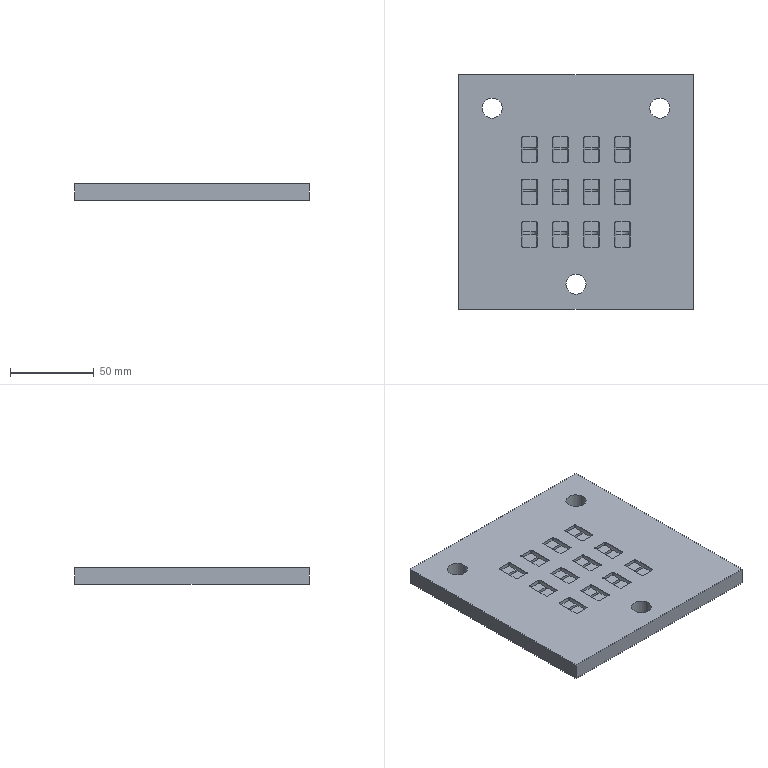CAM job | NX | mm | 3-axis | 1 set-up | 3 operations | part box 140 x 140 x 10
set-up 1
1. Z-Level Milling | Mill Mill5 D3 | ZLEVEL_PROFILE | path 0 mm | 0 min
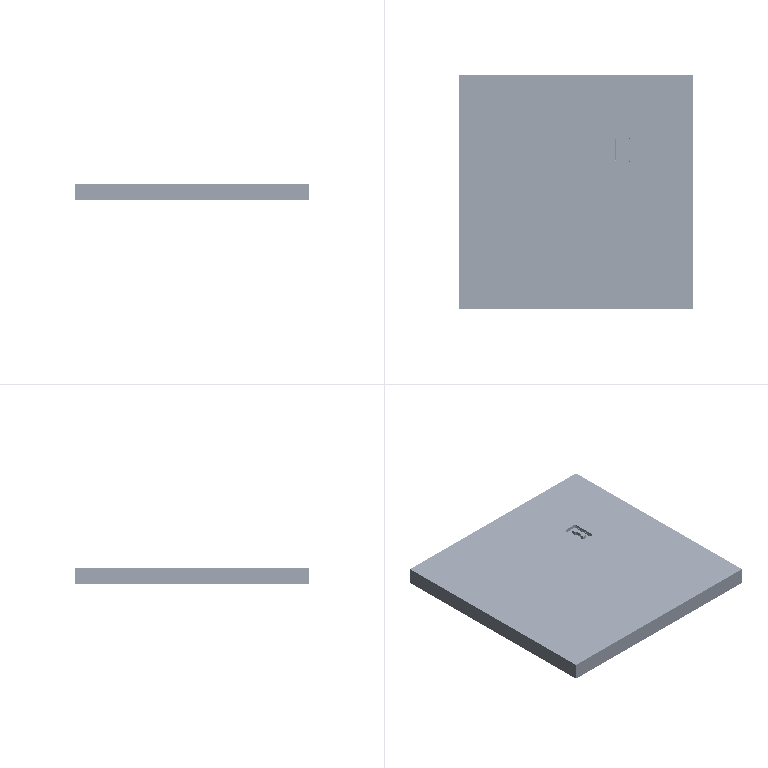2. Cavity Milling | Mill Mill5 D3 | CAVITY_MILL | path 0 mm | 0 min
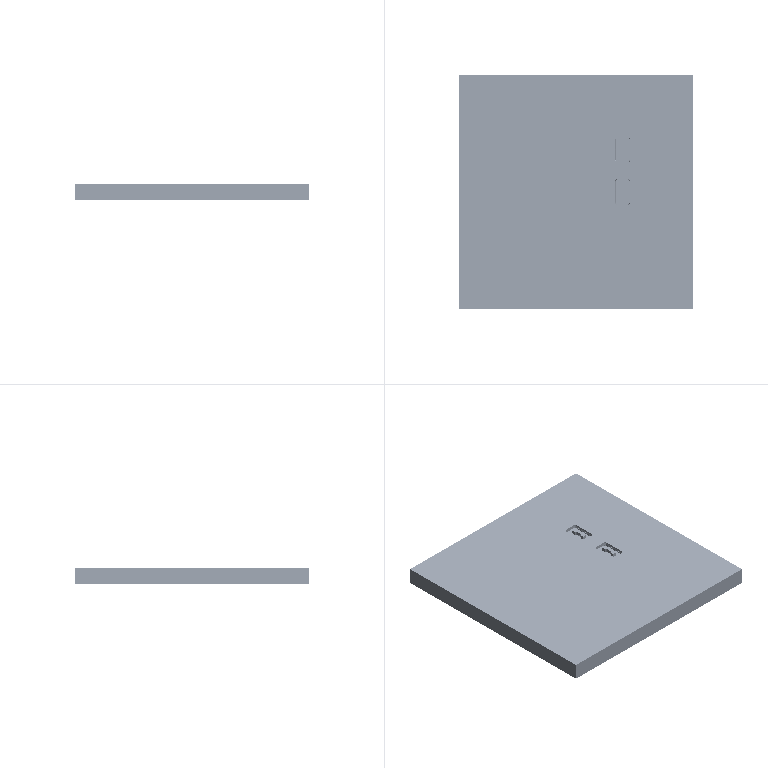3. Cavity Milling | Mill Mill5 D4 | CAVITY_MILL_1 | path 0 mm | 0 min